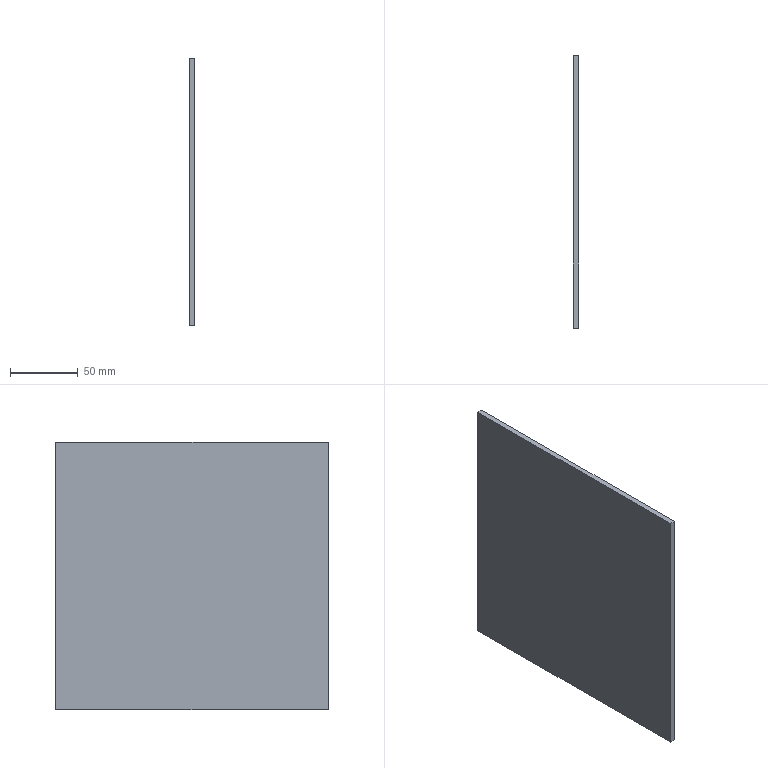Component | SolidWorks | Cover1-5-2XG1-1 | 1 solid | 6 faces | box 4 x 201 x 197 mm | volume 158388 mm3 | plane 6
build123d program:
from build123d import *

# Parameters (mm, degrees)
SKETCH3_W           = 201
SKETCH3_H           = 197
BOSS_EXTRUDE1_DEPTH = 4


with BuildPart() as part:
    # Sketch3 → Boss-Extrude1 (new body)
    with BuildSketch(Plane.XY):
        Rectangle(SKETCH3_W, SKETCH3_H)
    extrude(amount=BOSS_EXTRUDE1_DEPTH)


solid = part.part

# Placed as in the assembly
solid = solid.moved(Location((146.8, 0, 130), (90, -90, 0)))
STEP:
#1=COLOUR_RGB('',0.7922,0.8196,0.9333);
#2=FILL_AREA_STYLE_COLOUR('',#1);
#3=FILL_AREA_STYLE('',(#2));
#4=SURFACE_STYLE_FILL_AREA(#3);
#5=SURFACE_SIDE_STYLE('',(#4));
#6=SURFACE_STYLE_USAGE(.BOTH.,#5);
#7=PRESENTATION_STYLE_ASSIGNMENT((#6));
#8=CARTESIAN_POINT('',(5.78,3.957,8.996));
#9=VERTEX_POINT('',#8);
#10=CARTESIAN_POINT('',(5.78,3.957,1.24));
#11=VERTEX_POINT('',#10);
#12=CARTESIAN_POINT('',(5.78,3.957,8.996));
#13=DIRECTION('',(-0.,-0.,-1.));
#14=VECTOR('',#13,39.37);
#15=LINE('',#12,#14);
#16=EDGE_CURVE('',#9,#11,#15,.T.);
#17=ORIENTED_EDGE('',*,*,#16,.T.);
#18=CARTESIAN_POINT('',(5.622,3.957,1.24));
#19=VERTEX_POINT('',#18);
#20=CARTESIAN_POINT('',(5.622,3.957,1.24));
#21=DIRECTION('',(1.,-0.,-0.));
#22=VECTOR('',#21,39.37);
#23=LINE('',#20,#22);
#24=EDGE_CURVE('',#19,#11,#23,.T.);
#25=ORIENTED_EDGE('',*,*,#24,.F.);
#26=CARTESIAN_POINT('',(5.622,3.957,8.996));
#27=VERTEX_POINT('',#26);
#28=CARTESIAN_POINT('',(5.622,3.957,8.996));
#29=DIRECTION('',(-0.,-0.,-1.));
#30=VECTOR('',#29,39.37);
#31=LINE('',#28,#30);
#32=EDGE_CURVE('',#27,#19,#31,.T.);
#33=ORIENTED_EDGE('',*,*,#32,.F.);
#34=CARTESIAN_POINT('',(5.622,3.957,8.996));
#35=DIRECTION('',(1.,-0.,-0.));
#36=VECTOR('',#35,39.37);
#37=LINE('',#34,#36);
#38=EDGE_CURVE('',#27,#9,#37,.T.);
#39=ORIENTED_EDGE('',*,*,#38,.T.);
#40=EDGE_LOOP('',(#17,#25,#33,#39));
#41=FACE_OUTER_BOUND('',#40,.T.);
#42=CARTESIAN_POINT('',(5.622,3.957,8.996));
#43=DIRECTION('',(-0.,-1.,0.));
#44=DIRECTION('',(1.,-0.,-0.));
#45=AXIS2_PLACEMENT_3D('',#42,#43,#44);
#46=PLANE('',#45);
#47=ADVANCED_FACE('',(#41),#46,.F.);
#48=CARTESIAN_POINT('',(5.78,-3.957,1.24));
#49=VERTEX_POINT('',#48);
#50=CARTESIAN_POINT('',(5.78,3.957,1.24));
#51=DIRECTION('',(-0.,-1.,0.));
#52=VECTOR('',#51,39.37);
#53=LINE('',#50,#52);
#54=EDGE_CURVE('',#11,#49,#53,.T.);
#55=ORIENTED_EDGE('',*,*,#54,.T.);
#56=CARTESIAN_POINT('',(5.622,-3.957,1.24));
#57=VERTEX_POINT('',#56);
#58=CARTESIAN_POINT('',(5.622,-3.957,1.24));
#59=DIRECTION('',(1.,-0.,-0.));
#60=VECTOR('',#59,39.37);
#61=LINE('',#58,#60);
#62=EDGE_CURVE('',#57,#49,#61,.T.);
#63=ORIENTED_EDGE('',*,*,#62,.F.);
#64=CARTESIAN_POINT('',(5.622,3.957,1.24));
#65=DIRECTION('',(-0.,-1.,0.));
#66=VECTOR('',#65,39.37);
#67=LINE('',#64,#66);
#68=EDGE_CURVE('',#19,#57,#67,.T.);
#69=ORIENTED_EDGE('',*,*,#68,.F.);
#70=ORIENTED_EDGE('',*,*,#24,.T.);
#71=EDGE_LOOP('',(#55,#63,#69,#70));
#72=FACE_OUTER_BOUND('',#71,.T.);
#73=CARTESIAN_POINT('',(5.622,3.957,1.24));
#74=DIRECTION('',(0.,0.,1.));
#75=DIRECTION('',(-1.,0.,0.));
#76=AXIS2_PLACEMENT_3D('',#73,#74,#75);
#77=PLANE('',#76);
#78=ADVANCED_FACE('',(#72),#77,.F.);
#79=CARTESIAN_POINT('',(5.78,-3.957,8.996));
#80=VERTEX_POINT('',#79);
#81=CARTESIAN_POINT('',(5.78,-3.957,8.996));
#82=DIRECTION('',(0.,0.,1.));
#83=VECTOR('',#82,39.37);
#84=LINE('',#81,#83);
#85=EDGE_CURVE('',#49,#80,#84,.T.);
#86=ORIENTED_EDGE('',*,*,#85,.T.);
#87=CARTESIAN_POINT('',(5.622,-3.957,8.996));
#88=VERTEX_POINT('',#87);
#89=CARTESIAN_POINT('',(5.622,-3.957,8.996));
#90=DIRECTION('',(1.,-0.,-0.));
#91=VECTOR('',#90,39.37);
#92=LINE('',#89,#91);
#93=EDGE_CURVE('',#88,#80,#92,.T.);
#94=ORIENTED_EDGE('',*,*,#93,.F.);
#95=CARTESIAN_POINT('',(5.622,-3.957,8.996));
#96=DIRECTION('',(0.,0.,1.));
#97=VECTOR('',#96,39.37);
#98=LINE('',#95,#97);
#99=EDGE_CURVE('',#57,#88,#98,.T.);
#100=ORIENTED_EDGE('',*,*,#99,.F.);
#101=ORIENTED_EDGE('',*,*,#62,.T.);
#102=EDGE_LOOP('',(#86,#94,#100,#101));
#103=FACE_OUTER_BOUND('',#102,.T.);
#104=CARTESIAN_POINT('',(5.622,-3.957,8.996));
#105=DIRECTION('',(0.,1.,-0.));
#106=DIRECTION('',(-1.,0.,0.));
#107=AXIS2_PLACEMENT_3D('',#104,#105,#106);
#108=PLANE('',#107);
#109=ADVANCED_FACE('',(#103),#108,.F.);
#110=CARTESIAN_POINT('',(5.78,3.957,8.996));
#111=DIRECTION('',(0.,1.,-0.));
#112=VECTOR('',#111,39.37);
#113=LINE('',#110,#112);
#114=EDGE_CURVE('',#80,#9,#113,.T.);
#115=ORIENTED_EDGE('',*,*,#114,.T.);
#116=ORIENTED_EDGE('',*,*,#38,.F.);
#117=CARTESIAN_POINT('',(5.622,3.957,8.996));
#118=DIRECTION('',(0.,1.,-0.));
#119=VECTOR('',#118,39.37);
#120=LINE('',#117,#119);
#121=EDGE_CURVE('',#88,#27,#120,.T.);
#122=ORIENTED_EDGE('',*,*,#121,.F.);
#123=ORIENTED_EDGE('',*,*,#93,.T.);
#124=EDGE_LOOP('',(#115,#116,#122,#123));
#125=FACE_OUTER_BOUND('',#124,.T.);
#126=CARTESIAN_POINT('',(5.622,3.957,8.996));
#127=DIRECTION('',(-0.,-0.,-1.));
#128=DIRECTION('',(1.,-0.,-0.));
#129=AXIS2_PLACEMENT_3D('',#126,#127,#128);
#130=PLANE('',#129);
#131=ADVANCED_FACE('',(#125),#130,.F.);
#132=ORIENTED_EDGE('',*,*,#32,.T.);
#133=ORIENTED_EDGE('',*,*,#68,.T.);
#134=ORIENTED_EDGE('',*,*,#99,.T.);
#135=ORIENTED_EDGE('',*,*,#121,.T.);
#136=EDGE_LOOP('',(#132,#133,#134,#135));
#137=FACE_OUTER_BOUND('',#136,.T.);
#138=CARTESIAN_POINT('',(5.622,-0.,5.118));
#139=DIRECTION('',(-1.,0.,0.));
#140=DIRECTION('',(-0.,-1.,0.));
#141=AXIS2_PLACEMENT_3D('',#138,#139,#140);
#142=PLANE('',#141);
#143=ADVANCED_FACE('',(#137),#142,.T.);
#144=ORIENTED_EDGE('',*,*,#16,.F.);
#145=ORIENTED_EDGE('',*,*,#114,.F.);
#146=ORIENTED_EDGE('',*,*,#85,.F.);
#147=ORIENTED_EDGE('',*,*,#54,.F.);
#148=EDGE_LOOP('',(#144,#145,#146,#147));
#149=FACE_OUTER_BOUND('',#148,.T.);
#150=CARTESIAN_POINT('',(5.78,-0.,5.118));
#151=DIRECTION('',(-1.,0.,0.));
#152=DIRECTION('',(-0.,-1.,0.));
#153=AXIS2_PLACEMENT_3D('',#150,#151,#152);
#154=PLANE('',#153);
#155=ADVANCED_FACE('',(#149),#154,.F.);
#156=CLOSED_SHELL('',(#47,#78,#109,#131,#143,#155));
#157=MANIFOLD_SOLID_BREP('',#156);
#158=STYLED_ITEM('',(#7),#157);
#159=(LENGTH_UNIT()NAMED_UNIT(*)SI_UNIT($,.METRE.));
#160=LENGTH_MEASURE_WITH_UNIT(LENGTH_MEASURE(0.0254),#159);
#161=DIMENSIONAL_EXPONENTS(1.,0.,0.,0.,0.,0.,0.);
#162=(CONVERSION_BASED_UNIT('',#160)LENGTH_UNIT()NAMED_UNIT(#161));
#163=UNCERTAINTY_MEASURE_WITH_UNIT(LENGTH_MEASURE(0.00001),#162,'','');
#164=(NAMED_UNIT(*)PLANE_ANGLE_UNIT()SI_UNIT($,.RADIAN.));
#165=(NAMED_UNIT(*)SI_UNIT($,.STERADIAN.)SOLID_ANGLE_UNIT());
#166=(GEOMETRIC_REPRESENTATION_CONTEXT(3)GLOBAL_UNCERTAINTY_ASSIGNED_CONTEXT((#163))GLOBAL_UNIT_ASSIGNED_CONTEXT((#162,#164,#165))REPRESENTATION_CONTEXT('',''));
#167=MECHANICAL_DESIGN_GEOMETRIC_PRESENTATION_REPRESENTATION('',(#158),#166);
#168=PRESENTATION_LAYER_ASSIGNMENT('','',(#158));
#169=CARTESIAN_POINT('',(0.,0.,0.));
#170=DIRECTION('',(0.,0.,1.));
#171=DIRECTION('',(1.,0.,0.));
#172=AXIS2_PLACEMENT_3D('',#169,#170,#171);
#173=(LENGTH_UNIT()NAMED_UNIT(*)SI_UNIT($,.METRE.));
#174=LENGTH_MEASURE_WITH_UNIT(LENGTH_MEASURE(0.0254),#173);
#175=DIMENSIONAL_EXPONENTS(1.,0.,0.,0.,0.,0.,0.);
#176=(CONVERSION_BASED_UNIT('',#174)LENGTH_UNIT()NAMED_UNIT(#175));
#177=UNCERTAINTY_MEASURE_WITH_UNIT(LENGTH_MEASURE(0.00001),#176,'','');
#178=(NAMED_UNIT(*)PLANE_ANGLE_UNIT()SI_UNIT($,.RADIAN.));
#179=(NAMED_UNIT(*)SI_UNIT($,.STERADIAN.)SOLID_ANGLE_UNIT());
#180=(GEOMETRIC_REPRESENTATION_CONTEXT(3)GLOBAL_UNCERTAINTY_ASSIGNED_CONTEXT((#177))GLOBAL_UNIT_ASSIGNED_CONTEXT((#176,#178,#179))REPRESENTATION_CONTEXT('',''));
#181=ADVANCED_BREP_SHAPE_REPRESENTATION('',(#157,#172),#180);